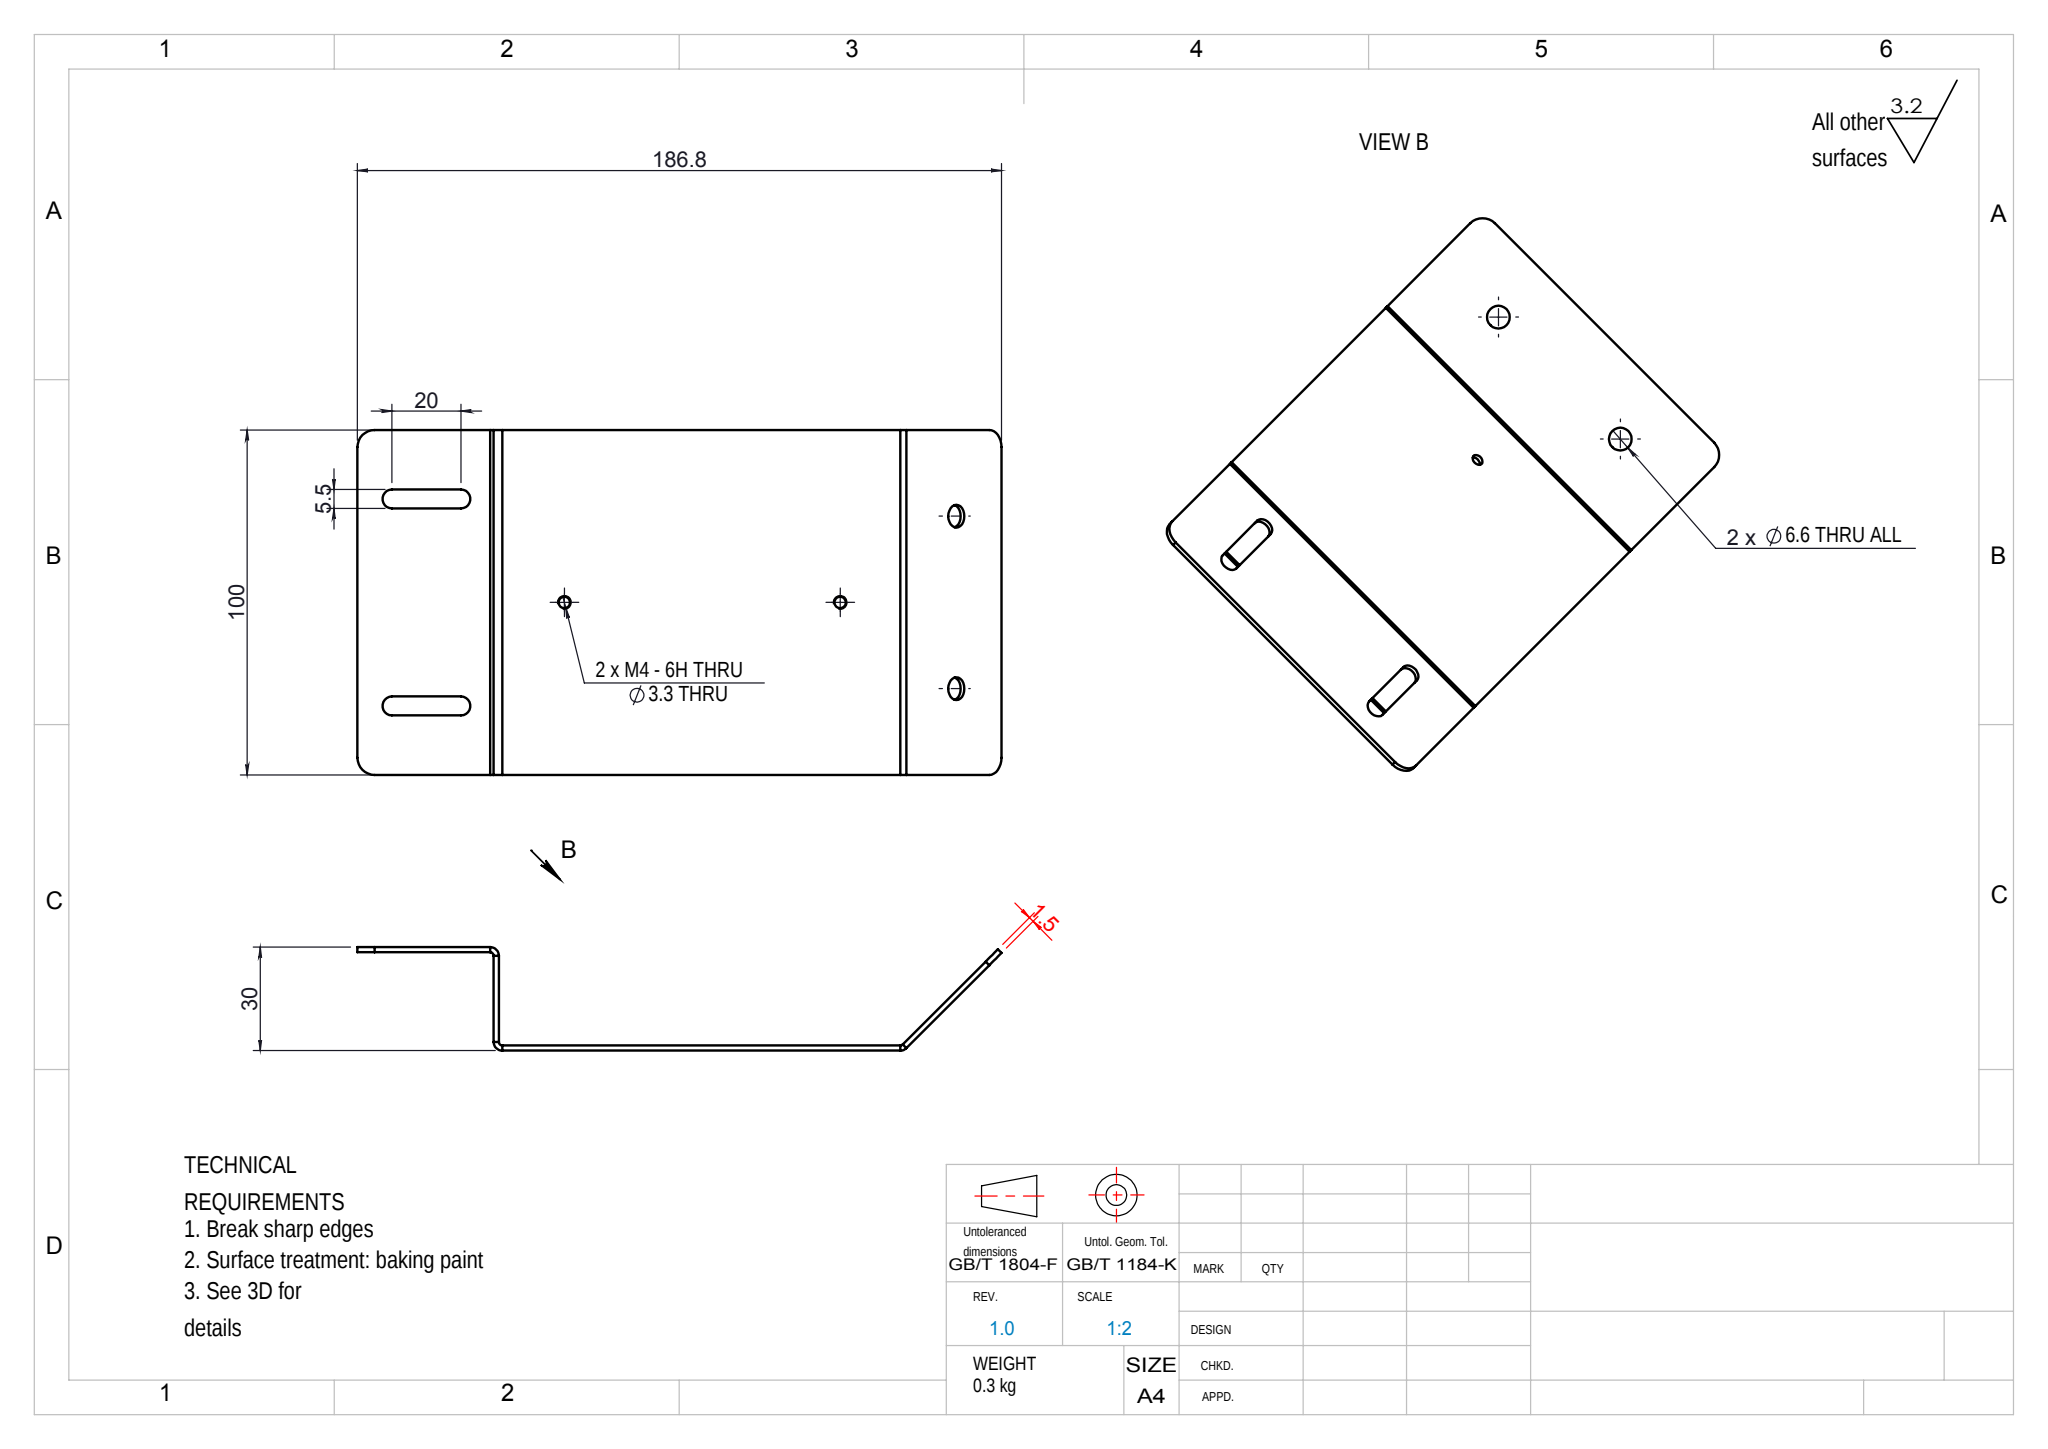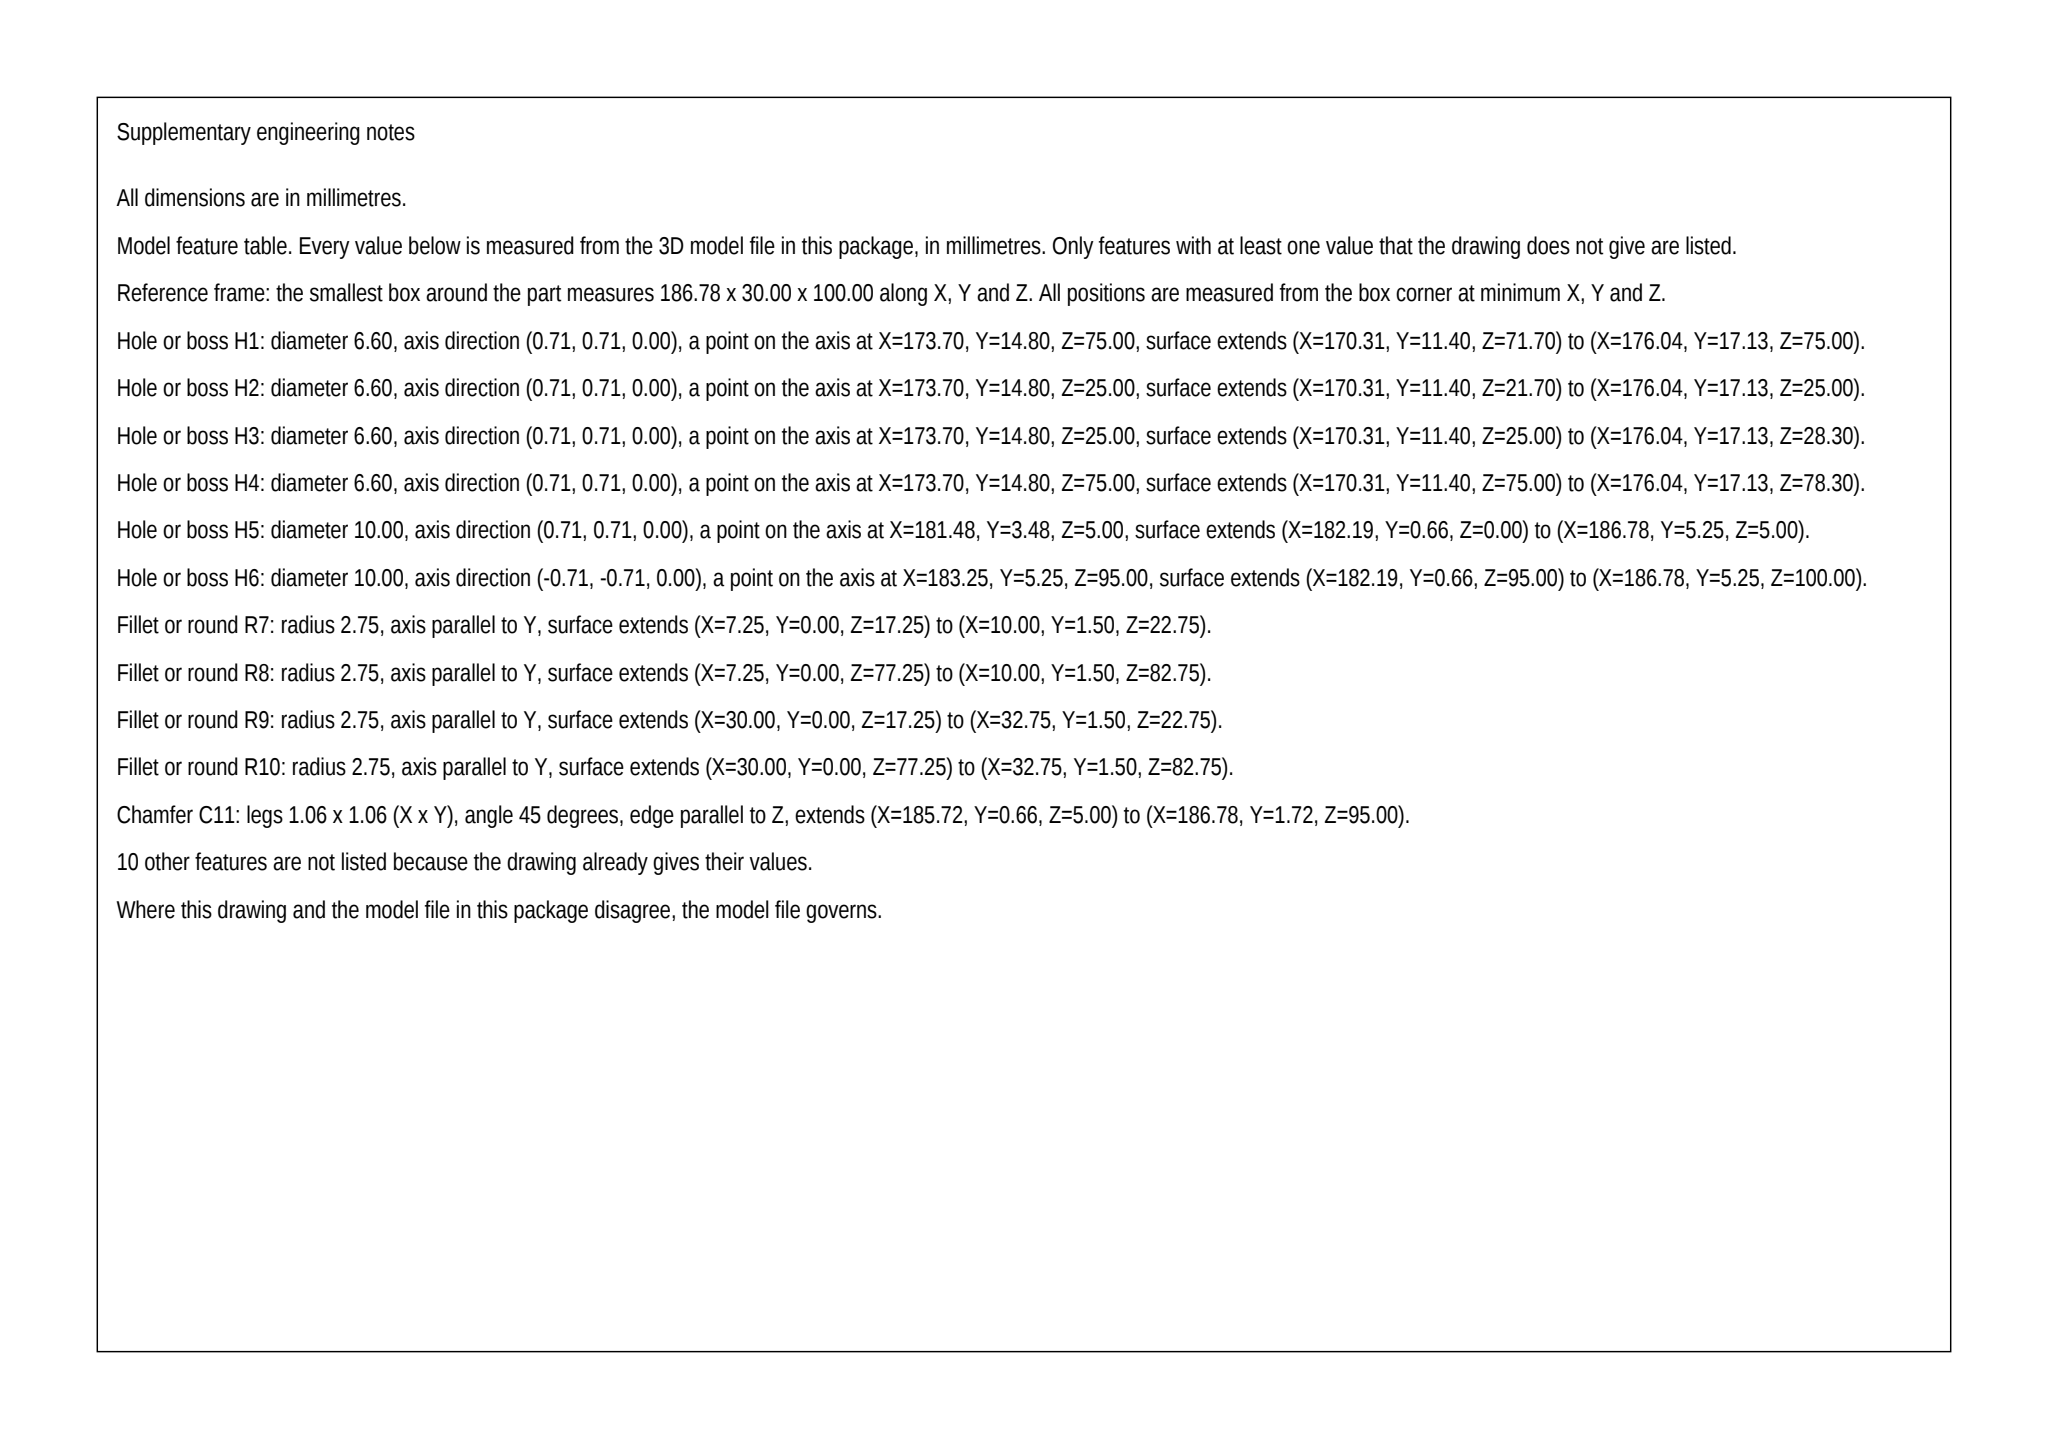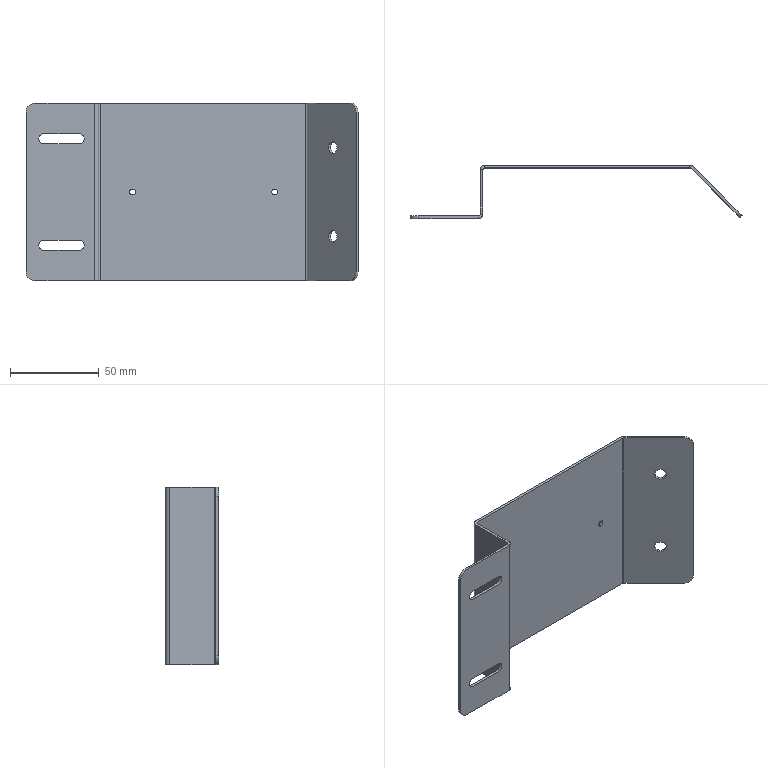Part | SolidWorks | mm | 1 solid | 50 faces | box 186.78 x 30 x 100 mm | volume 33158 mm3 | plane 28 | cylinder 22 | commonest cylinder face diameters 3.3 x4 6.6 x4 5.5 x4 10 x4 5 x3 2 x3
Drawing notes:
2 X M4-6H THRU (TAP DRILL Ø3.3 THRU), HOLE AXES NORMAL TO FLAT FACE, LOCATED 60 AND 140 FROM LEFT EDGE, 50 FROM BOTTOM EDGE | from the solid: cylinders dia 3.3, axis y, pos [60,-,50] and [140,-,50], length 1.5
2 X SLOT 5.5 WIDE X 20 LONG (END RADII CENTRES 10 AND 30 FROM LEFT EDGE), SLOT CENTRELINES 20 AND 80 FROM BOTTOM EDGE, THRU 1.5 THK | from the solid: cylinders dia 5.5, axis y, pos [10,-,20],[10,-,80],[30,-,20],[30,-,80], length 1.5
2 X Ø6.6 FULLY THRU VERTICAL FLANGE, AXES PARALLEL TO LENGTH, LOCATED 25 AND 75 FROM BOTTOM EDGE, 14.8 ABOVE FLAT BASE FACE | from the solid: cylinders dia 6.6, axis x, pos [-,14.8,25] and [-,14.8,75]
2 X Ø10 CORNER RELIEF HOLE THRU FLAT, CENTRES 5 FROM LEFT EDGE, 5 AND 95 FROM BOTTOM EDGE | from the solid: cylinders dia 10, axis y, pos [5,-,5] and [5,-,95], length 1.5
2 X Ø10 RELIEF IN VERTICAL FLANGE, AXES PARALLEL TO LENGTH, CENTRES 5 AND 95 FROM BOTTOM EDGE AT 3.48 AND 5.25 ABOVE FLAT BASE FACE | from the solid: cylinders dia 10, axis x, pos [-,3.48,5] and [-,5.25,95], length 4.6
VERTICAL FLANGE BEND: INNER BEND FACE AT 39.5, OUTER FACE AT 41.0 FROM LEFT EDGE (MATERIAL 1.5 THK) | from the solid: axis_planes x=39.5 and x=41.0; y planes 0/1.5 give 1.5 thickness
ANGLED END FLANGE BEND LINE LOCATED 157.46 FROM LEFT EDGE (BEND RELIEF FEATURE ON BEND LINE) | from the solid: cylinders dia 2.0/5.0, axis z, pos x=157.46 (bend relief on bend line)
BEND RELIEF NOTCHES ON VERTICAL FLANGE BEND LINE AT X=38.5 AND X=42.0 (Ø5 WITH Ø2 END), THRU FULL 100 WIDTH DIRECTION | from the solid: cylinders dia 2.0/5.0, axis z, pos [38.5,2.5] and [42.0,27.5]
OVERALL PART ENVELOPE 186.784 X 100 X 30; ALL DIMENSIONS IN MILLIMETRES | from the solid: bbox_xyz [186.784, 30.0, 100.0], STEP units mm
ALL DIMENSIONS IN MILLIMETERS (mm) | from the solid: STEP bbox_xyz 186.784 x 30.0 x 100.0 mm
SHEET THICKNESS 1.5 | from the solid: axis_planes normal y at 0.0 and 1.5 (and 28.5/30.0)
2X M4 TAPPED THRU (Ø3.3 PILOT) IN FLAT PANEL, AT X=60 AND X=140 FROM LEFT EDGE, Z=50 FROM BOTTOM EDGE | from the solid: cylinders dia 3.3, axis y, pos (60,-,50) and (140,-,50), length 1.5
2X SLOT 5.5 WIDE, END CENTERS AT X=10 AND X=30 FROM LEFT EDGE (20 BETWEEN CENTERS), SLOT CENTERLINES AT Z=20 AND Z=80 FROM BOTTOM EDGE, THRU | from the solid: cylinders dia 5.5, axis y, pos (10,-,20)(30,-,20)(10,-,80)(30,-,80), length 1.5; planes z 17.25/22.75/77.25/82.75
2X Ø6.6 THRU ANGLED END FLANGE, AT Z=25 AND Z=75 FROM BOTTOM EDGE, HOLE AXIS HEIGHT Y=14.8 FROM BASE | from the solid: cylinders dia 6.6, axis x, pos (-,14.8,25) and (-,14.8,75), length 5.73
2X Ø10 CORNER RELIEF HOLE THRU FLAT PANEL AT X=5, Z=5 AND X=5, Z=95 FROM LEFT/BOTTOM EDGES | from the solid: cylinders dia 10.0, axis y, pos (5,-,5) and (5,-,95), length 1.5
2X Ø10 RELIEF IN END FLANGE, AXIS ALONG X, AT Z=5 / Y=3.48 AND Z=95 / Y=5.25 | from the solid: cylinders dia 10.0, axis x, pos (-,3.48,5) and (-,5.25,95), length 4.6
ALL FORMED BENDS: INSIDE R1.0, OUTSIDE R2.5 | from the solid: cylinders dia 2.0 and dia 5.0, axis z, length 100.0 (concentric pairs)
VERTICAL WEB FACES AT X=39.5 AND X=41.0 FROM LEFT EDGE; BEND AXES AT X=38.5 / Y=2.5 AND X=42.0 / Y=27.5 | from the solid: axis_planes normal x at 39.5 and 41.0; cylinders axis z at (38.5,2.5) and (42.0,27.5)
BEND AXIS OF INCLINED END FLANGE AT X=157.46 FROM LEFT EDGE (Y=27.5) | from the solid: cylinders dia 2.0/5.0, axis z, pos (157.46,27.5), length 100.0
2X M4-6H TAPPED THRU (Ø3.3 PILOT) IN FLAT PANEL, 1.5 THK, AT X=60 AND X=140 FROM LEFT EDGE, Z=50 FROM BOTTOM EDGE | from the solid: cylinders dia 3.3, axis y, at [60,null,50] and [140,null,50], length 1.5
BEND RELIEF ON ANGLED END FLANGE BEND LINE AT X=157.46 FROM LEFT EDGE: Ø5 WITH Ø2 END, AXES ALONG WIDTH (Z), THRU FULL 100 WIDTH | from the solid: cylinders dia 5.0 and dia 2.0, axis z, at [157.46,27.5], length 100
INCLINED END FLANGE EXTENDS FROM BEND AXIS X=157.46 TO X=186.784 FROM LEFT EDGE (29.32 HORIZONTAL PROJECTION) | from the solid: bbox_xyz x=186.784 and bend axis cylinders at x=157.46
Ø6.6 HOLES IN INCLINED END FLANGE: AXES PARALLEL TO X, HOLE PATH LENGTH 5.73 THROUGH 1.5 THK MATERIAL, AT Z=25 AND Z=75 FROM BOTTOM EDGE, Y=14.8 ABOVE BASE | from the solid: cylinders dia 6.6, axis x, at [null,14.8,25] and [null,14.8,75], length 5.73
2X M4-6H TAPPED THRU (Ø3.3 PILOT) IN 1.5 THK FLAT PANEL, HOLE AXES NORMAL TO PANEL, AT X=60 AND X=140 FROM LEFT EDGE, Z=50 FROM BOTTOM EDGE | from the solid: cylinders dia 3.3, axis y, at [60,null,50] and [140,null,50], length 1.5 (2 each); planes y=0 / y=1.5
INCLINED END FLANGE BENT 45° TO FLAT BASE FACE (BEND AXIS AT X=157.46 FROM LEFT EDGE, Y=27.5 ABOVE BASE); FLANGE RISES 45° IN BOTH X AND Y, FULL 100 WIDTH | from the solid: inclined_planes angle_to_xyz_axes [45.0,45.0,90.0], bbox_from [158.2,0.7,0.0], size [27.6,27.6,100.0]; convex arc Ø5 / concave arc Ø2 at z-axis pos (157.5,27.5), arc_deg 45
2X M4-6H TAPPED THRU (Ø3.3 PILOT) IN 1.5 THK FLAT PANEL, AXES NORMAL TO PANEL, AT X=60 AND X=140 FROM LEFT EDGE, Z=50 FROM BOTTOM EDGE | from the solid: hole/bore dia 3.3, axis y, at (60,50) and (140,50), from y=28.5 to y=30.0
2X M4-6H TAPPED THRU (Ø3.3 PILOT) IN FLAT PANEL, AXES NORMAL TO PANEL, AT X=60 AND X=140 FROM LEFT EDGE, Z=50 FROM BOTTOM EDGE | from the solid: cylinders: hole/bore Ø3.3, axis y, at (60,50) and (140,50), from y=28.5 to y=30.0
MATERIAL THICKNESS 1.5 (FLAT PANEL FACES AT Y=0.0 AND Y=1.5) | from the solid: axis_planes: y=0.0 and y=1.5 over x[0,38.5], z[0,100]; also y=28.5 and y=30.0 base faces